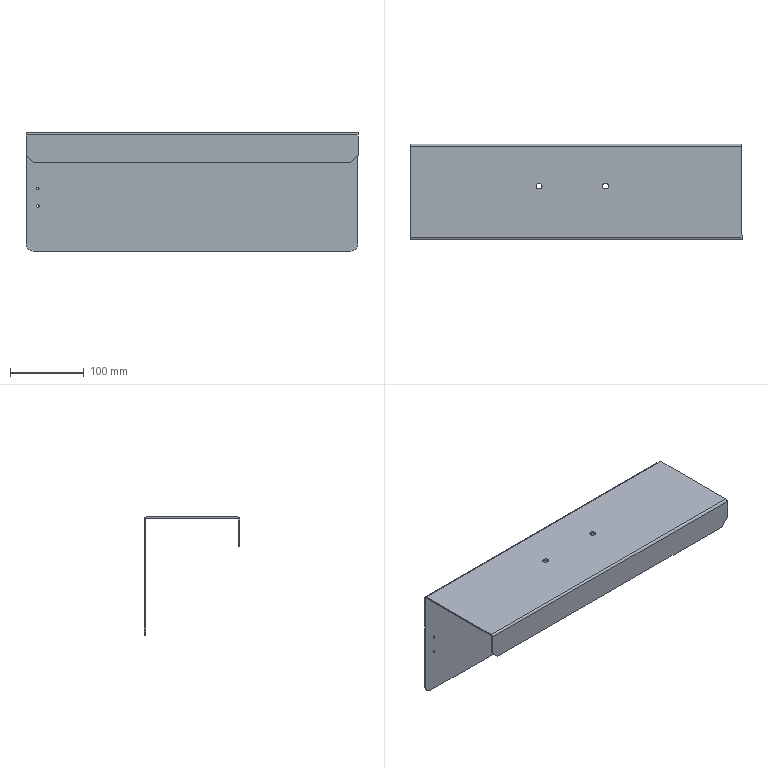Component | SolidWorks | -UpperGuard-1 | 1 solid | 34 faces | box 450 x 130 x 160 mm | volume 291537 mm3 | plane 20 | cylinder 14 | commonest cylinder face diameters 3.3 x4 8 x4 5.473 x2 1.473 x2 20 x2
STEP:
#1=COLOUR_RGB('',0.7922,0.8196,0.9333);
#2=FILL_AREA_STYLE_COLOUR('',#1);
#3=FILL_AREA_STYLE('',(#2));
#4=SURFACE_STYLE_FILL_AREA(#3);
#5=SURFACE_SIDE_STYLE('',(#4));
#6=SURFACE_STYLE_USAGE(.BOTH.,#5);
#7=PRESENTATION_STYLE_ASSIGNMENT((#6));
#8=CARTESIAN_POINT('',(-6.85,51.555,3.951));
#9=VERTEX_POINT('',#8);
#10=CARTESIAN_POINT('',(-6.85,51.555,4.081));
#11=VERTEX_POINT('',#10);
#12=CARTESIAN_POINT('',(-6.85,51.555,4.016));
#13=DIRECTION('',(-0.,1.,0.));
#14=DIRECTION('',(0.,0.,1.));
#15=AXIS2_PLACEMENT_3D('',#12,#13,#14);
#16=CIRCLE('',#15,0.06496);
#17=EDGE_CURVE('',#9,#11,#16,.T.);
#18=ORIENTED_EDGE('',*,*,#17,.F.);
#19=CARTESIAN_POINT('',(-6.85,51.634,3.951));
#20=VERTEX_POINT('',#19);
#21=CARTESIAN_POINT('',(-6.85,51.634,3.951));
#22=DIRECTION('',(-0.,1.,0.));
#23=VECTOR('',#22,39.37);
#24=LINE('',#21,#23);
#25=EDGE_CURVE('',#9,#20,#24,.T.);
#26=ORIENTED_EDGE('',*,*,#25,.T.);
#27=CARTESIAN_POINT('',(-6.85,51.634,4.081));
#28=VERTEX_POINT('',#27);
#29=CARTESIAN_POINT('',(-6.85,51.634,4.016));
#30=DIRECTION('',(-0.,1.,0.));
#31=DIRECTION('',(0.,0.,1.));
#32=AXIS2_PLACEMENT_3D('',#29,#30,#31);
#33=CIRCLE('',#32,0.06496);
#34=EDGE_CURVE('',#20,#28,#33,.T.);
#35=ORIENTED_EDGE('',*,*,#34,.T.);
#36=CARTESIAN_POINT('',(-6.85,51.634,4.081));
#37=DIRECTION('',(-0.,1.,0.));
#38=VECTOR('',#37,39.37);
#39=LINE('',#36,#38);
#40=EDGE_CURVE('',#11,#28,#39,.T.);
#41=ORIENTED_EDGE('',*,*,#40,.F.);
#42=EDGE_LOOP('',(#18,#26,#35,#41));
#43=FACE_OUTER_BOUND('',#42,.T.);
#44=CARTESIAN_POINT('',(-6.85,51.634,4.016));
#45=DIRECTION('',(-0.,1.,0.));
#46=DIRECTION('',(0.,0.,1.));
#47=AXIS2_PLACEMENT_3D('',#44,#45,#46);
#48=CYLINDRICAL_SURFACE('',#47,0.06496);
#49=ADVANCED_FACE('',(#43),#48,.F.);
#50=CARTESIAN_POINT('',(-6.85,51.555,3.006));
#51=VERTEX_POINT('',#50);
#52=CARTESIAN_POINT('',(-6.85,51.555,3.136));
#53=VERTEX_POINT('',#52);
#54=CARTESIAN_POINT('',(-6.85,51.555,3.071));
#55=DIRECTION('',(-0.,1.,0.));
#56=DIRECTION('',(0.,0.,1.));
#57=AXIS2_PLACEMENT_3D('',#54,#55,#56);
#58=CIRCLE('',#57,0.06496);
#59=EDGE_CURVE('',#51,#53,#58,.T.);
#60=ORIENTED_EDGE('',*,*,#59,.F.);
#61=CARTESIAN_POINT('',(-6.85,51.634,3.006));
#62=VERTEX_POINT('',#61);
#63=CARTESIAN_POINT('',(-6.85,51.634,3.006));
#64=DIRECTION('',(-0.,1.,0.));
#65=VECTOR('',#64,39.37);
#66=LINE('',#63,#65);
#67=EDGE_CURVE('',#51,#62,#66,.T.);
#68=ORIENTED_EDGE('',*,*,#67,.T.);
#69=CARTESIAN_POINT('',(-6.85,51.634,3.136));
#70=VERTEX_POINT('',#69);
#71=CARTESIAN_POINT('',(-6.85,51.634,3.071));
#72=DIRECTION('',(-0.,1.,0.));
#73=DIRECTION('',(0.,0.,1.));
#74=AXIS2_PLACEMENT_3D('',#71,#72,#73);
#75=CIRCLE('',#74,0.06496);
#76=EDGE_CURVE('',#62,#70,#75,.T.);
#77=ORIENTED_EDGE('',*,*,#76,.T.);
#78=CARTESIAN_POINT('',(-6.85,51.634,3.136));
#79=DIRECTION('',(-0.,1.,0.));
#80=VECTOR('',#79,39.37);
#81=LINE('',#78,#80);
#82=EDGE_CURVE('',#53,#70,#81,.T.);
#83=ORIENTED_EDGE('',*,*,#82,.F.);
#84=EDGE_LOOP('',(#60,#68,#77,#83));
#85=FACE_OUTER_BOUND('',#84,.T.);
#86=CARTESIAN_POINT('',(-6.85,51.634,3.071));
#87=DIRECTION('',(-0.,1.,0.));
#88=DIRECTION('',(0.,0.,1.));
#89=AXIS2_PLACEMENT_3D('',#86,#87,#88);
#90=CYLINDRICAL_SURFACE('',#89,0.06496);
#91=ADVANCED_FACE('',(#85),#90,.F.);
#92=CARTESIAN_POINT('',(-0.4331,49.39,6.89));
#93=VERTEX_POINT('',#92);
#94=CARTESIAN_POINT('',(-0.748,49.39,6.89));
#95=VERTEX_POINT('',#94);
#96=CARTESIAN_POINT('',(-0.5906,49.39,6.89));
#97=DIRECTION('',(0.,-0.,1.));
#98=DIRECTION('',(-1.,0.,0.));
#99=AXIS2_PLACEMENT_3D('',#96,#97,#98);
#100=CIRCLE('',#99,0.1575);
#101=EDGE_CURVE('',#93,#95,#100,.T.);
#102=ORIENTED_EDGE('',*,*,#101,.F.);
#103=CARTESIAN_POINT('',(-0.4331,49.39,6.969));
#104=VERTEX_POINT('',#103);
#105=CARTESIAN_POINT('',(-0.4331,49.39,6.575));
#106=DIRECTION('',(0.,-0.,1.));
#107=VECTOR('',#106,39.37);
#108=LINE('',#105,#107);
#109=EDGE_CURVE('',#93,#104,#108,.T.);
#110=ORIENTED_EDGE('',*,*,#109,.T.);
#111=CARTESIAN_POINT('',(-0.748,49.39,6.969));
#112=VERTEX_POINT('',#111);
#113=CARTESIAN_POINT('',(-0.5906,49.39,6.969));
#114=DIRECTION('',(0.,-0.,1.));
#115=DIRECTION('',(-1.,0.,0.));
#116=AXIS2_PLACEMENT_3D('',#113,#114,#115);
#117=CIRCLE('',#116,0.1575);
#118=EDGE_CURVE('',#104,#112,#117,.T.);
#119=ORIENTED_EDGE('',*,*,#118,.T.);
#120=CARTESIAN_POINT('',(-0.748,49.39,6.575));
#121=DIRECTION('',(0.,-0.,1.));
#122=VECTOR('',#121,39.37);
#123=LINE('',#120,#122);
#124=EDGE_CURVE('',#95,#112,#123,.T.);
#125=ORIENTED_EDGE('',*,*,#124,.F.);
#126=EDGE_LOOP('',(#102,#110,#119,#125));
#127=FACE_OUTER_BOUND('',#126,.T.);
#128=CARTESIAN_POINT('',(-0.5906,49.39,6.575));
#129=DIRECTION('',(0.,-0.,1.));
#130=DIRECTION('',(-1.,0.,0.));
#131=AXIS2_PLACEMENT_3D('',#128,#129,#130);
#132=CYLINDRICAL_SURFACE('',#131,0.1575);
#133=ADVANCED_FACE('',(#127),#132,.F.);
#134=CARTESIAN_POINT('',(3.11,49.39,6.89));
#135=VERTEX_POINT('',#134);
#136=CARTESIAN_POINT('',(2.795,49.39,6.89));
#137=VERTEX_POINT('',#136);
#138=CARTESIAN_POINT('',(2.953,49.39,6.89));
#139=DIRECTION('',(0.,-0.,1.));
#140=DIRECTION('',(-1.,0.,0.));
#141=AXIS2_PLACEMENT_3D('',#138,#139,#140);
#142=CIRCLE('',#141,0.1575);
#143=EDGE_CURVE('',#135,#137,#142,.T.);
#144=ORIENTED_EDGE('',*,*,#143,.F.);
#145=CARTESIAN_POINT('',(3.11,49.39,6.969));
#146=VERTEX_POINT('',#145);
#147=CARTESIAN_POINT('',(3.11,49.39,6.575));
#148=DIRECTION('',(0.,-0.,1.));
#149=VECTOR('',#148,39.37);
#150=LINE('',#147,#149);
#151=EDGE_CURVE('',#135,#146,#150,.T.);
#152=ORIENTED_EDGE('',*,*,#151,.T.);
#153=CARTESIAN_POINT('',(2.795,49.39,6.969));
#154=VERTEX_POINT('',#153);
#155=CARTESIAN_POINT('',(2.953,49.39,6.969));
#156=DIRECTION('',(0.,-0.,1.));
#157=DIRECTION('',(-1.,0.,0.));
#158=AXIS2_PLACEMENT_3D('',#155,#156,#157);
#159=CIRCLE('',#158,0.1575);
#160=EDGE_CURVE('',#146,#154,#159,.T.);
#161=ORIENTED_EDGE('',*,*,#160,.T.);
#162=CARTESIAN_POINT('',(2.795,49.39,6.575));
#163=DIRECTION('',(0.,-0.,1.));
#164=VECTOR('',#163,39.37);
#165=LINE('',#162,#164);
#166=EDGE_CURVE('',#137,#154,#165,.T.);
#167=ORIENTED_EDGE('',*,*,#166,.F.);
#168=EDGE_LOOP('',(#144,#152,#161,#167));
#169=FACE_OUTER_BOUND('',#168,.T.);
#170=CARTESIAN_POINT('',(2.953,49.39,6.575));
#171=DIRECTION('',(0.,-0.,1.));
#172=DIRECTION('',(-1.,0.,0.));
#173=AXIS2_PLACEMENT_3D('',#170,#171,#172);
#174=CYLINDRICAL_SURFACE('',#173,0.1575);
#175=ADVANCED_FACE('',(#169),#174,.F.);
#176=CARTESIAN_POINT('',(10.236,51.634,6.861));
#177=VERTEX_POINT('',#176);
#178=CARTESIAN_POINT('',(10.236,51.555,6.861));
#179=VERTEX_POINT('',#178);
#180=CARTESIAN_POINT('',(10.236,51.634,6.861));
#181=DIRECTION('',(0.,-1.,-0.));
#182=VECTOR('',#181,39.37);
#183=LINE('',#180,#182);
#184=EDGE_CURVE('',#177,#179,#183,.T.);
#185=ORIENTED_EDGE('',*,*,#184,.F.);
#186=CARTESIAN_POINT('',(10.236,51.526,6.969));
#187=VERTEX_POINT('',#186);
#188=CARTESIAN_POINT('',(10.236,51.526,6.861));
#189=DIRECTION('',(-1.,-0.,-0.));
#190=DIRECTION('',(0.,0.,1.));
#191=AXIS2_PLACEMENT_3D('',#188,#189,#190);
#192=CIRCLE('',#191,0.1077);
#193=EDGE_CURVE('',#187,#177,#192,.T.);
#194=ORIENTED_EDGE('',*,*,#193,.F.);
#195=CARTESIAN_POINT('',(10.236,51.526,6.89));
#196=VERTEX_POINT('',#195);
#197=CARTESIAN_POINT('',(10.236,51.526,6.89));
#198=DIRECTION('',(0.,-0.,1.));
#199=VECTOR('',#198,39.37);
#200=LINE('',#197,#199);
#201=EDGE_CURVE('',#196,#187,#200,.T.);
#202=ORIENTED_EDGE('',*,*,#201,.F.);
#203=CARTESIAN_POINT('',(10.236,51.526,6.861));
#204=DIRECTION('',(-1.,-0.,-0.));
#205=DIRECTION('',(0.,0.,1.));
#206=AXIS2_PLACEMENT_3D('',#203,#204,#205);
#207=CIRCLE('',#206,0.029);
#208=EDGE_CURVE('',#196,#179,#207,.T.);
#209=ORIENTED_EDGE('',*,*,#208,.T.);
#210=EDGE_LOOP('',(#185,#194,#202,#209));
#211=FACE_OUTER_BOUND('',#210,.T.);
#212=CARTESIAN_POINT('',(10.236,51.634,6.861));
#213=DIRECTION('',(1.,0.,-0.));
#214=DIRECTION('',(0.,-0.,1.));
#215=AXIS2_PLACEMENT_3D('',#212,#213,#214);
#216=PLANE('',#215);
#217=ADVANCED_FACE('',(#211),#216,.T.);
#218=CARTESIAN_POINT('',(10.236,51.555,1.063));
#219=VERTEX_POINT('',#218);
#220=CARTESIAN_POINT('',(10.236,51.555,6.969));
#221=DIRECTION('',(-0.,0.,-1.));
#222=VECTOR('',#221,39.37);
#223=LINE('',#220,#222);
#224=EDGE_CURVE('',#179,#219,#223,.T.);
#225=ORIENTED_EDGE('',*,*,#224,.T.);
#226=CARTESIAN_POINT('',(10.236,51.634,1.063));
#227=VERTEX_POINT('',#226);
#228=CARTESIAN_POINT('',(10.236,51.526,1.063));
#229=DIRECTION('',(-0.,1.,0.));
#230=VECTOR('',#229,39.37);
#231=LINE('',#228,#230);
#232=EDGE_CURVE('',#219,#227,#231,.T.);
#233=ORIENTED_EDGE('',*,*,#232,.T.);
#234=CARTESIAN_POINT('',(10.236,51.634,6.969));
#235=DIRECTION('',(-0.,0.,-1.));
#236=VECTOR('',#235,39.37);
#237=LINE('',#234,#236);
#238=EDGE_CURVE('',#177,#227,#237,.T.);
#239=ORIENTED_EDGE('',*,*,#238,.F.);
#240=ORIENTED_EDGE('',*,*,#184,.T.);
#241=EDGE_LOOP('',(#225,#233,#239,#240));
#242=FACE_OUTER_BOUND('',#241,.T.);
#243=CARTESIAN_POINT('',(10.236,51.526,6.89));
#244=DIRECTION('',(1.,0.,-0.));
#245=DIRECTION('',(0.,-0.,1.));
#246=AXIS2_PLACEMENT_3D('',#243,#244,#245);
#247=PLANE('',#246);
#248=ADVANCED_FACE('',(#242),#247,.T.);
#249=CARTESIAN_POINT('',(-7.48,51.526,6.969));
#250=VERTEX_POINT('',#249);
#251=CARTESIAN_POINT('',(-7.48,51.526,6.89));
#252=VERTEX_POINT('',#251);
#253=CARTESIAN_POINT('',(-7.48,51.526,6.969));
#254=DIRECTION('',(-0.,0.,-1.));
#255=VECTOR('',#254,39.37);
#256=LINE('',#253,#255);
#257=EDGE_CURVE('',#250,#252,#256,.T.);
#258=ORIENTED_EDGE('',*,*,#257,.F.);
#259=CARTESIAN_POINT('',(-7.48,51.634,6.861));
#260=VERTEX_POINT('',#259);
#261=CARTESIAN_POINT('',(-7.48,51.526,6.861));
#262=DIRECTION('',(-1.,-0.,-0.));
#263=DIRECTION('',(0.,0.,1.));
#264=AXIS2_PLACEMENT_3D('',#261,#262,#263);
#265=CIRCLE('',#264,0.1077);
#266=EDGE_CURVE('',#250,#260,#265,.T.);
#267=ORIENTED_EDGE('',*,*,#266,.T.);
#268=CARTESIAN_POINT('',(-7.48,51.555,6.861));
#269=VERTEX_POINT('',#268);
#270=CARTESIAN_POINT('',(-7.48,51.555,6.861));
#271=DIRECTION('',(-0.,1.,0.));
#272=VECTOR('',#271,39.37);
#273=LINE('',#270,#272);
#274=EDGE_CURVE('',#269,#260,#273,.T.);
#275=ORIENTED_EDGE('',*,*,#274,.F.);
#276=CARTESIAN_POINT('',(-7.48,51.526,6.861));
#277=DIRECTION('',(-1.,-0.,-0.));
#278=DIRECTION('',(0.,0.,1.));
#279=AXIS2_PLACEMENT_3D('',#276,#277,#278);
#280=CIRCLE('',#279,0.029);
#281=EDGE_CURVE('',#252,#269,#280,.T.);
#282=ORIENTED_EDGE('',*,*,#281,.F.);
#283=EDGE_LOOP('',(#258,#267,#275,#282));
#284=FACE_OUTER_BOUND('',#283,.T.);
#285=CARTESIAN_POINT('',(-7.48,51.526,6.969));
#286=DIRECTION('',(-1.,-0.,0.));
#287=DIRECTION('',(-0.,0.,-1.));
#288=AXIS2_PLACEMENT_3D('',#285,#286,#287);
#289=PLANE('',#288);
#290=ADVANCED_FACE('',(#284),#289,.T.);
#291=CARTESIAN_POINT('',(-7.48,46.623,6.969));
#292=VERTEX_POINT('',#291);
#293=CARTESIAN_POINT('',(-7.48,46.713,6.969));
#294=DIRECTION('',(-0.,1.,0.));
#295=VECTOR('',#294,39.37);
#296=LINE('',#293,#295);
#297=EDGE_CURVE('',#292,#250,#296,.T.);
#298=ORIENTED_EDGE('',*,*,#297,.T.);
#299=ORIENTED_EDGE('',*,*,#257,.T.);
#300=CARTESIAN_POINT('',(-7.48,46.623,6.89));
#301=VERTEX_POINT('',#300);
#302=CARTESIAN_POINT('',(-7.48,46.713,6.89));
#303=DIRECTION('',(-0.,1.,0.));
#304=VECTOR('',#303,39.37);
#305=LINE('',#302,#304);
#306=EDGE_CURVE('',#301,#252,#305,.T.);
#307=ORIENTED_EDGE('',*,*,#306,.F.);
#308=CARTESIAN_POINT('',(-7.48,46.623,6.89));
#309=DIRECTION('',(0.,-0.,1.));
#310=VECTOR('',#309,39.37);
#311=LINE('',#308,#310);
#312=EDGE_CURVE('',#301,#292,#311,.T.);
#313=ORIENTED_EDGE('',*,*,#312,.T.);
#314=EDGE_LOOP('',(#298,#299,#307,#313));
#315=FACE_OUTER_BOUND('',#314,.T.);
#316=CARTESIAN_POINT('',(-7.48,51.555,6.861));
#317=DIRECTION('',(-1.,-0.,0.));
#318=DIRECTION('',(-0.,0.,-1.));
#319=AXIS2_PLACEMENT_3D('',#316,#317,#318);
#320=PLANE('',#319);
#321=ADVANCED_FACE('',(#315),#320,.T.);
#322=CARTESIAN_POINT('',(-6.85,51.555,4.016));
#323=DIRECTION('',(-0.,1.,0.));
#324=DIRECTION('',(0.,0.,1.));
#325=AXIS2_PLACEMENT_3D('',#322,#323,#324);
#326=CIRCLE('',#325,0.06496);
#327=EDGE_CURVE('',#11,#9,#326,.T.);
#328=ORIENTED_EDGE('',*,*,#327,.T.);
#329=ORIENTED_EDGE('',*,*,#17,.T.);
#330=EDGE_LOOP('',(#328,#329));
#331=FACE_BOUND('',#330,.T.);
#332=CARTESIAN_POINT('',(-6.85,51.555,3.071));
#333=DIRECTION('',(-0.,1.,0.));
#334=DIRECTION('',(0.,0.,1.));
#335=AXIS2_PLACEMENT_3D('',#332,#333,#334);
#336=CIRCLE('',#335,0.06496);
#337=EDGE_CURVE('',#53,#51,#336,.T.);
#338=ORIENTED_EDGE('',*,*,#337,.T.);
#339=ORIENTED_EDGE('',*,*,#59,.T.);
#340=EDGE_LOOP('',(#338,#339));
#341=FACE_BOUND('',#340,.T.);
#342=CARTESIAN_POINT('',(-7.48,51.555,1.063));
#343=VERTEX_POINT('',#342);
#344=CARTESIAN_POINT('',(-7.48,51.555,6.969));
#345=DIRECTION('',(-0.,0.,-1.));
#346=VECTOR('',#345,39.37);
#347=LINE('',#344,#346);
#348=EDGE_CURVE('',#269,#343,#347,.T.);
#349=ORIENTED_EDGE('',*,*,#348,.T.);
#350=CARTESIAN_POINT('',(-7.087,51.555,0.6693));
#351=VERTEX_POINT('',#350);
#352=CARTESIAN_POINT('',(-7.087,51.555,1.063));
#353=DIRECTION('',(0.,-1.,-0.));
#354=DIRECTION('',(0.,0.,1.));
#355=AXIS2_PLACEMENT_3D('',#352,#353,#354);
#356=CIRCLE('',#355,0.3937);
#357=EDGE_CURVE('',#343,#351,#356,.T.);
#358=ORIENTED_EDGE('',*,*,#357,.T.);
#359=CARTESIAN_POINT('',(9.843,51.555,0.6693));
#360=VERTEX_POINT('',#359);
#361=CARTESIAN_POINT('',(10.236,51.555,0.6693));
#362=DIRECTION('',(-1.,-0.,-0.));
#363=VECTOR('',#362,39.37);
#364=LINE('',#361,#363);
#365=EDGE_CURVE('',#360,#351,#364,.T.);
#366=ORIENTED_EDGE('',*,*,#365,.F.);
#367=CARTESIAN_POINT('',(9.843,51.555,1.063));
#368=DIRECTION('',(0.,-1.,-0.));
#369=DIRECTION('',(0.,0.,1.));
#370=AXIS2_PLACEMENT_3D('',#367,#368,#369);
#371=CIRCLE('',#370,0.3937);
#372=EDGE_CURVE('',#360,#219,#371,.T.);
#373=ORIENTED_EDGE('',*,*,#372,.T.);
#374=ORIENTED_EDGE('',*,*,#224,.F.);
#375=CARTESIAN_POINT('',(10.236,51.555,6.861));
#376=DIRECTION('',(-1.,-0.,-0.));
#377=VECTOR('',#376,39.37);
#378=LINE('',#375,#377);
#379=EDGE_CURVE('',#179,#269,#378,.T.);
#380=ORIENTED_EDGE('',*,*,#379,.T.);
#381=EDGE_LOOP('',(#349,#358,#366,#373,#374,#380));
#382=FACE_OUTER_BOUND('',#381,.T.);
#383=CARTESIAN_POINT('',(10.236,51.555,6.969));
#384=DIRECTION('',(-0.,1.,0.));
#385=DIRECTION('',(0.,-0.,1.));
#386=AXIS2_PLACEMENT_3D('',#383,#384,#385);
#387=PLANE('',#386);
#388=ADVANCED_FACE('',(#331,#341,#382),#387,.F.);
#389=ORIENTED_EDGE('',*,*,#365,.T.);
#390=CARTESIAN_POINT('',(-7.087,51.634,0.6693));
#391=VERTEX_POINT('',#390);
#392=CARTESIAN_POINT('',(-7.087,51.634,0.6693));
#393=DIRECTION('',(-0.,1.,0.));
#394=VECTOR('',#393,39.37);
#395=LINE('',#392,#394);
#396=EDGE_CURVE('',#351,#391,#395,.T.);
#397=ORIENTED_EDGE('',*,*,#396,.T.);
#398=CARTESIAN_POINT('',(9.843,51.634,0.6693));
#399=VERTEX_POINT('',#398);
#400=CARTESIAN_POINT('',(10.236,51.634,0.6693));
#401=DIRECTION('',(-1.,-0.,-0.));
#402=VECTOR('',#401,39.37);
#403=LINE('',#400,#402);
#404=EDGE_CURVE('',#399,#391,#403,.T.);
#405=ORIENTED_EDGE('',*,*,#404,.F.);
#406=CARTESIAN_POINT('',(9.843,51.634,0.6693));
#407=DIRECTION('',(0.,-1.,-0.));
#408=VECTOR('',#407,39.37);
#409=LINE('',#406,#408);
#410=EDGE_CURVE('',#399,#360,#409,.T.);
#411=ORIENTED_EDGE('',*,*,#410,.T.);
#412=EDGE_LOOP('',(#389,#397,#405,#411));
#413=FACE_OUTER_BOUND('',#412,.T.);
#414=CARTESIAN_POINT('',(10.236,51.634,0.6693));
#415=DIRECTION('',(0.,0.,-1.));
#416=DIRECTION('',(1.,0.,0.));
#417=AXIS2_PLACEMENT_3D('',#414,#415,#416);
#418=PLANE('',#417);
#419=ADVANCED_FACE('',(#413),#418,.T.);
#420=CARTESIAN_POINT('',(-6.85,51.634,4.016));
#421=DIRECTION('',(-0.,1.,0.));
#422=DIRECTION('',(0.,0.,1.));
#423=AXIS2_PLACEMENT_3D('',#420,#421,#422);
#424=CIRCLE('',#423,0.06496);
#425=EDGE_CURVE('',#28,#20,#424,.T.);
#426=ORIENTED_EDGE('',*,*,#425,.F.);
#427=ORIENTED_EDGE('',*,*,#34,.F.);
#428=EDGE_LOOP('',(#426,#427));
#429=FACE_BOUND('',#428,.T.);
#430=CARTESIAN_POINT('',(-6.85,51.634,3.071));
#431=DIRECTION('',(-0.,1.,0.));
#432=DIRECTION('',(0.,0.,1.));
#433=AXIS2_PLACEMENT_3D('',#430,#431,#432);
#434=CIRCLE('',#433,0.06496);
#435=EDGE_CURVE('',#70,#62,#434,.T.);
#436=ORIENTED_EDGE('',*,*,#435,.F.);
#437=ORIENTED_EDGE('',*,*,#76,.F.);
#438=EDGE_LOOP('',(#436,#437));
#439=FACE_BOUND('',#438,.T.);
#440=ORIENTED_EDGE('',*,*,#404,.T.);
#441=CARTESIAN_POINT('',(-7.48,51.634,1.063));
#442=VERTEX_POINT('',#441);
#443=CARTESIAN_POINT('',(-7.087,51.634,1.063));
#444=DIRECTION('',(-0.,1.,0.));
#445=DIRECTION('',(0.,0.,1.));
#446=AXIS2_PLACEMENT_3D('',#443,#444,#445);
#447=CIRCLE('',#446,0.3937);
#448=EDGE_CURVE('',#391,#442,#447,.T.);
#449=ORIENTED_EDGE('',*,*,#448,.T.);
#450=CARTESIAN_POINT('',(-7.48,51.634,6.969));
#451=DIRECTION('',(-0.,0.,-1.));
#452=VECTOR('',#451,39.37);
#453=LINE('',#450,#452);
#454=EDGE_CURVE('',#260,#442,#453,.T.);
#455=ORIENTED_EDGE('',*,*,#454,.F.);
#456=CARTESIAN_POINT('',(10.236,51.634,6.861));
#457=DIRECTION('',(-1.,-0.,-0.));
#458=VECTOR('',#457,39.37);
#459=LINE('',#456,#458);
#460=EDGE_CURVE('',#177,#260,#459,.T.);
#461=ORIENTED_EDGE('',*,*,#460,.F.);
#462=ORIENTED_EDGE('',*,*,#238,.T.);
#463=CARTESIAN_POINT('',(9.843,51.634,1.063));
#464=DIRECTION('',(-0.,1.,0.));
#465=DIRECTION('',(0.,0.,1.));
#466=AXIS2_PLACEMENT_3D('',#463,#464,#465);
#467=CIRCLE('',#466,0.3937);
#468=EDGE_CURVE('',#227,#399,#467,.T.);
#469=ORIENTED_EDGE('',*,*,#468,.T.);
#470=EDGE_LOOP('',(#440,#449,#455,#461,#462,#469));
#471=FACE_OUTER_BOUND('',#470,.T.);
#472=CARTESIAN_POINT('',(10.236,51.634,6.969));
#473=DIRECTION('',(-0.,1.,0.));
#474=DIRECTION('',(0.,-0.,1.));
#475=AXIS2_PLACEMENT_3D('',#472,#473,#474);
#476=PLANE('',#475);
#477=ADVANCED_FACE('',(#429,#439,#471),#476,.T.);
#478=ORIENTED_EDGE('',*,*,#266,.F.);
#479=CARTESIAN_POINT('',(10.236,51.526,6.969));
#480=DIRECTION('',(-1.,-0.,-0.));
#481=VECTOR('',#480,39.37);
#482=LINE('',#479,#481);
#483=EDGE_CURVE('',#187,#250,#482,.T.);
#484=ORIENTED_EDGE('',*,*,#483,.F.);
#485=ORIENTED_EDGE('',*,*,#193,.T.);
#486=ORIENTED_EDGE('',*,*,#460,.T.);
#487=EDGE_LOOP('',(#478,#484,#485,#486));
#488=FACE_OUTER_BOUND('',#487,.T.);
#489=CARTESIAN_POINT('',(10.236,51.526,6.861));
#490=DIRECTION('',(-1.,-0.,-0.));
#491=DIRECTION('',(0.,0.,-1.));
#492=AXIS2_PLACEMENT_3D('',#489,#490,#491);
#493=CYLINDRICAL_SURFACE('',#492,0.1077);
#494=ADVANCED_FACE('',(#488),#493,.T.);
#495=CARTESIAN_POINT('',(-0.5906,49.39,6.969));
#496=DIRECTION('',(0.,-0.,1.));
#497=DIRECTION('',(-1.,0.,0.));
#498=AXIS2_PLACEMENT_3D('',#495,#496,#497);
#499=CIRCLE('',#498,0.1575);
#500=EDGE_CURVE('',#112,#104,#499,.T.);
#501=ORIENTED_EDGE('',*,*,#500,.F.);
#502=ORIENTED_EDGE('',*,*,#118,.F.);
#503=EDGE_LOOP('',(#501,#502));
#504=FACE_BOUND('',#503,.T.);
#505=CARTESIAN_POINT('',(2.953,49.39,6.969));
#506=DIRECTION('',(0.,-0.,1.));
#507=DIRECTION('',(-1.,0.,0.));
#508=AXIS2_PLACEMENT_3D('',#505,#506,#507);
#509=CIRCLE('',#508,0.1575);
#510=EDGE_CURVE('',#154,#146,#509,.T.);
#511=ORIENTED_EDGE('',*,*,#510,.F.);
#512=ORIENTED_EDGE('',*,*,#160,.F.);
#513=EDGE_LOOP('',(#511,#512));
#514=FACE_BOUND('',#513,.T.);
#515=ORIENTED_EDGE('',*,*,#297,.F.);
#516=CARTESIAN_POINT('',(10.236,46.623,6.969));
#517=VERTEX_POINT('',#516);
#518=CARTESIAN_POINT('',(-7.48,46.623,6.969));
#519=DIRECTION('',(1.,0.,0.));
#520=VECTOR('',#519,39.37);
#521=LINE('',#518,#520);
#522=EDGE_CURVE('',#292,#517,#521,.T.);
#523=ORIENTED_EDGE('',*,*,#522,.T.);
#524=CARTESIAN_POINT('',(10.236,46.713,6.969));
#525=DIRECTION('',(-0.,1.,0.));
#526=VECTOR('',#525,39.37);
#527=LINE('',#524,#526);
#528=EDGE_CURVE('',#517,#187,#527,.T.);
#529=ORIENTED_EDGE('',*,*,#528,.T.);
#530=ORIENTED_EDGE('',*,*,#483,.T.);
#531=EDGE_LOOP('',(#515,#523,#529,#530));
#532=FACE_OUTER_BOUND('',#531,.T.);
#533=CARTESIAN_POINT('',(10.236,46.713,6.969));
#534=DIRECTION('',(-0.,-0.,1.));
#535=DIRECTION('',(-1.,-0.,-0.));
#536=AXIS2_PLACEMENT_3D('',#533,#534,#535);
#537=PLANE('',#536);
#538=ADVANCED_FACE('',(#504,#514,#532),#537,.T.);
#539=CARTESIAN_POINT('',(-0.5906,49.39,6.89));
#540=DIRECTION('',(0.,-0.,1.));
#541=DIRECTION('',(-1.,0.,0.));
#542=AXIS2_PLACEMENT_3D('',#539,#540,#541);
#543=CIRCLE('',#542,0.1575);
#544=EDGE_CURVE('',#95,#93,#543,.T.);
#545=ORIENTED_EDGE('',*,*,#544,.T.);
#546=ORIENTED_EDGE('',*,*,#101,.T.);
#547=EDGE_LOOP('',(#545,#546));
#548=FACE_BOUND('',#547,.T.);
#549=CARTESIAN_POINT('',(2.953,49.39,6.89));
#550=DIRECTION('',(0.,-0.,1.));
#551=DIRECTION('',(-1.,0.,0.));
#552=AXIS2_PLACEMENT_3D('',#549,#550,#551);
#553=CIRCLE('',#552,0.1575);
#554=EDGE_CURVE('',#137,#135,#553,.T.);
#555=ORIENTED_EDGE('',*,*,#554,.T.);
#556=ORIENTED_EDGE('',*,*,#143,.T.);
#557=EDGE_LOOP('',(#555,#556));
#558=FACE_BOUND('',#557,.T.);
#559=ORIENTED_EDGE('',*,*,#306,.T.);
#560=CARTESIAN_POINT('',(10.236,51.526,6.89));
#561=DIRECTION('',(-1.,-0.,-0.));
#562=VECTOR('',#561,39.37);
#563=LINE('',#560,#562);
#564=EDGE_CURVE('',#196,#252,#563,.T.);
#565=ORIENTED_EDGE('',*,*,#564,.F.);
#566=CARTESIAN_POINT('',(10.236,46.623,6.89));
#567=VERTEX_POINT('',#566);
#568=CARTESIAN_POINT('',(10.236,46.713,6.89));
#569=DIRECTION('',(-0.,1.,0.));
#570=VECTOR('',#569,39.37);
#571=LINE('',#568,#570);
#572=EDGE_CURVE('',#567,#196,#571,.T.);
#573=ORIENTED_EDGE('',*,*,#572,.F.);
#574=CARTESIAN_POINT('',(-7.48,46.623,6.89));
#575=DIRECTION('',(1.,0.,0.));
#576=VECTOR('',#575,39.37);
#577=LINE('',#574,#576);
#578=EDGE_CURVE('',#301,#567,#577,.T.);
#579=ORIENTED_EDGE('',*,*,#578,.F.);
#580=EDGE_LOOP('',(#559,#565,#573,#579));
#581=FACE_OUTER_BOUND('',#580,.T.);
#582=CARTESIAN_POINT('',(10.236,46.713,6.89));
#583=DIRECTION('',(-0.,-0.,1.));
#584=DIRECTION('',(-1.,-0.,-0.));
#585=AXIS2_PLACEMENT_3D('',#582,#583,#584);
#586=PLANE('',#585);
#587=ADVANCED_FACE('',(#548,#558,#581),#586,.F.);
#588=ORIENTED_EDGE('',*,*,#281,.T.);
#589=ORIENTED_EDGE('',*,*,#379,.F.);
#590=ORIENTED_EDGE('',*,*,#208,.F.);
#591=ORIENTED_EDGE('',*,*,#564,.T.);
#592=EDGE_LOOP('',(#588,#589,#590,#591));
#593=FACE_OUTER_BOUND('',#592,.T.);
#594=CARTESIAN_POINT('',(10.236,51.526,6.861));
#595=DIRECTION('',(-1.,-0.,-0.));
#596=DIRECTION('',(0.,0.,-1.));
#597=AXIS2_PLACEMENT_3D('',#594,#595,#596);
#598=CYLINDRICAL_SURFACE('',#597,0.029);
#599=ADVANCED_FACE('',(#593),#598,.F.);
#600=ORIENTED_EDGE('',*,*,#572,.T.);
#601=ORIENTED_EDGE('',*,*,#201,.T.);
#602=ORIENTED_EDGE('',*,*,#528,.F.);
#603=CARTESIAN_POINT('',(10.236,46.623,6.89));
#604=DIRECTION('',(0.,-0.,1.));
#605=VECTOR('',#604,39.37);
#606=LINE('',#603,#605);
#607=EDGE_CURVE('',#567,#517,#606,.T.);
#608=ORIENTED_EDGE('',*,*,#607,.F.);
#609=EDGE_LOOP('',(#600,#601,#602,#608));
#610=FACE_OUTER_BOUND('',#609,.T.);
#611=CARTESIAN_POINT('',(10.236,51.526,6.861));
#612=DIRECTION('',(1.,0.,-0.));
#613=DIRECTION('',(0.,-0.,1.));
#614=AXIS2_PLACEMENT_3D('',#611,#612,#613);
#615=PLANE('',#614);
#616=ADVANCED_FACE('',(#610),#615,.T.);
#617=ORIENTED_EDGE('',*,*,#454,.T.);
#618=CARTESIAN_POINT('',(-7.48,51.555,1.063));
#619=DIRECTION('',(0.,-1.,-0.));
#620=VECTOR('',#619,39.37);
#621=LINE('',#618,#620);
#622=EDGE_CURVE('',#442,#343,#621,.T.);
#623=ORIENTED_EDGE('',*,*,#622,.T.);
#624=ORIENTED_EDGE('',*,*,#348,.F.);
#625=ORIENTED_EDGE('',*,*,#274,.T.);
#626=EDGE_LOOP('',(#617,#623,#624,#625));
#627=FACE_OUTER_BOUND('',#626,.T.);
#628=CARTESIAN_POINT('',(-7.48,51.526,6.861));
#629=DIRECTION('',(1.,0.,-0.));
#630=DIRECTION('',(0.,-0.,1.));
#631=AXIS2_PLACEMENT_3D('',#628,#629,#630);
#632=PLANE('',#631);
#633=ADVANCED_FACE('',(#627),#632,.F.);
#634=ORIENTED_EDGE('',*,*,#151,.F.);
#635=ORIENTED_EDGE('',*,*,#554,.F.);
#636=ORIENTED_EDGE('',*,*,#166,.T.);
#637=ORIENTED_EDGE('',*,*,#510,.T.);
#638=EDGE_LOOP('',(#634,#635,#636,#637));
#639=FACE_OUTER_BOUND('',#638,.T.);
#640=CARTESIAN_POINT('',(2.953,49.39,6.575));
#641=DIRECTION('',(0.,-0.,1.));
#642=DIRECTION('',(-1.,0.,0.));
#643=AXIS2_PLACEMENT_3D('',#640,#641,#642);
#644=CYLINDRICAL_SURFACE('',#643,0.1575);
#645=ADVANCED_FACE('',(#639),#644,.F.);
#646=ORIENTED_EDGE('',*,*,#109,.F.);
#647=ORIENTED_EDGE('',*,*,#544,.F.);
#648=ORIENTED_EDGE('',*,*,#124,.T.);
#649=ORIENTED_EDGE('',*,*,#500,.T.);
#650=EDGE_LOOP('',(#646,#647,#648,#649));
#651=FACE_OUTER_BOUND('',#650,.T.);
#652=CARTESIAN_POINT('',(-0.5906,49.39,6.575));
#653=DIRECTION('',(0.,-0.,1.));
#654=DIRECTION('',(-1.,0.,0.));
#655=AXIS2_PLACEMENT_3D('',#652,#653,#654);
#656=CYLINDRICAL_SURFACE('',#655,0.1575);
#657=ADVANCED_FACE('',(#651),#656,.F.);
#658=ORIENTED_EDGE('',*,*,#448,.F.);
#659=ORIENTED_EDGE('',*,*,#396,.F.);
#660=ORIENTED_EDGE('',*,*,#357,.F.);
#661=ORIENTED_EDGE('',*,*,#622,.F.);
#662=EDGE_LOOP('',(#658,#659,#660,#661));
#663=FACE_OUTER_BOUND('',#662,.T.);
#664=CARTESIAN_POINT('',(-7.087,51.526,1.063));
#665=DIRECTION('',(-0.,1.,0.));
#666=DIRECTION('',(0.,0.,1.));
#667=AXIS2_PLACEMENT_3D('',#664,#665,#666);
#668=CYLINDRICAL_SURFACE('',#667,0.3937);
#669=ADVANCED_FACE('',(#663),#668,.T.);
#670=ORIENTED_EDGE('',*,*,#468,.F.);
#671=ORIENTED_EDGE('',*,*,#232,.F.);
#672=ORIENTED_EDGE('',*,*,#372,.F.);
#673=ORIENTED_EDGE('',*,*,#410,.F.);
#674=EDGE_LOOP('',(#670,#671,#672,#673));
#675=FACE_OUTER_BOUND('',#674,.T.);
#676=CARTESIAN_POINT('',(9.843,51.634,1.063));
#677=DIRECTION('',(0.,-1.,-0.));
#678=DIRECTION('',(0.,0.,-1.));
#679=AXIS2_PLACEMENT_3D('',#676,#677,#678);
#680=CYLINDRICAL_SURFACE('',#679,0.3937);
#681=ADVANCED_FACE('',(#675),#680,.T.);
#682=ORIENTED_EDGE('',*,*,#67,.F.);
#683=ORIENTED_EDGE('',*,*,#337,.F.);
#684=ORIENTED_EDGE('',*,*,#82,.T.);
#685=ORIENTED_EDGE('',*,*,#435,.T.);
#686=EDGE_LOOP('',(#682,#683,#684,#685));
#687=FACE_OUTER_BOUND('',#686,.T.);
#688=CARTESIAN_POINT('',(-6.85,51.634,3.071));
#689=DIRECTION('',(-0.,1.,0.));
#690=DIRECTION('',(0.,0.,1.));
#691=AXIS2_PLACEMENT_3D('',#688,#689,#690);
#692=CYLINDRICAL_SURFACE('',#691,0.06496);
#693=ADVANCED_FACE('',(#687),#692,.F.);
#694=ORIENTED_EDGE('',*,*,#25,.F.);
#695=ORIENTED_EDGE('',*,*,#327,.F.);
#696=ORIENTED_EDGE('',*,*,#40,.T.);
#697=ORIENTED_EDGE('',*,*,#425,.T.);
#698=EDGE_LOOP('',(#694,#695,#696,#697));
#699=FACE_OUTER_BOUND('',#698,.T.);
#700=CARTESIAN_POINT('',(-6.85,51.634,4.016));
#701=DIRECTION('',(-0.,1.,0.));
#702=DIRECTION('',(0.,0.,1.));
#703=AXIS2_PLACEMENT_3D('',#700,#701,#702);
#704=CYLINDRICAL_SURFACE('',#703,0.06496);
#705=ADVANCED_FACE('',(#699),#704,.F.);
#706=CARTESIAN_POINT('',(10.236,46.594,6.861));
#707=VERTEX_POINT('',#706);
#708=CARTESIAN_POINT('',(10.236,46.516,6.861));
#709=VERTEX_POINT('',#708);
#710=CARTESIAN_POINT('',(10.236,46.516,6.861));
#711=DIRECTION('',(0.,-1.,0.));
#712=VECTOR('',#711,39.37);
#713=LINE('',#710,#712);
#714=EDGE_CURVE('',#707,#709,#713,.T.);
#715=ORIENTED_EDGE('',*,*,#714,.F.);
#716=CARTESIAN_POINT('',(10.236,46.623,6.861));
#717=DIRECTION('',(1.,0.,0.));
#718=DIRECTION('',(0.,0.,-1.));
#719=AXIS2_PLACEMENT_3D('',#716,#717,#718);
#720=CIRCLE('',#719,0.029);
#721=EDGE_CURVE('',#567,#707,#720,.T.);
#722=ORIENTED_EDGE('',*,*,#721,.F.);
#723=ORIENTED_EDGE('',*,*,#607,.T.);
#724=CARTESIAN_POINT('',(10.236,46.623,6.861));
#725=DIRECTION('',(1.,0.,0.));
#726=DIRECTION('',(0.,0.,-1.));
#727=AXIS2_PLACEMENT_3D('',#724,#725,#726);
#728=CIRCLE('',#727,0.1077);
#729=EDGE_CURVE('',#517,#709,#728,.T.);
#730=ORIENTED_EDGE('',*,*,#729,.T.);
#731=EDGE_LOOP('',(#715,#722,#723,#730));
#732=FACE_OUTER_BOUND('',#731,.T.);
#733=CARTESIAN_POINT('',(10.236,46.623,6.861));
#734=DIRECTION('',(1.,0.,-0.));
#735=DIRECTION('',(0.,-0.,1.));
#736=AXIS2_PLACEMENT_3D('',#733,#734,#735);
#737=PLANE('',#736);
#738=ADVANCED_FACE('',(#732),#737,.T.);
#739=CARTESIAN_POINT('',(-7.48,46.594,6.861));
#740=VERTEX_POINT('',#739);
#741=CARTESIAN_POINT('',(-7.48,46.623,6.861));
#742=DIRECTION('',(-1.,-0.,-0.));
#743=DIRECTION('',(0.,0.,-1.));
#744=AXIS2_PLACEMENT_3D('',#741,#742,#743);
#745=CIRCLE('',#744,0.029);
#746=EDGE_CURVE('',#740,#301,#745,.T.);
#747=ORIENTED_EDGE('',*,*,#746,.F.);
#748=CARTESIAN_POINT('',(-7.48,46.516,6.861));
#749=VERTEX_POINT('',#748);
#750=CARTESIAN_POINT('',(-7.48,46.594,6.861));
#751=DIRECTION('',(0.,-1.,0.));
#752=VECTOR('',#751,39.37);
#753=LINE('',#750,#752);
#754=EDGE_CURVE('',#740,#749,#753,.T.);
#755=ORIENTED_EDGE('',*,*,#754,.T.);
#756=CARTESIAN_POINT('',(-7.48,46.623,6.861));
#757=DIRECTION('',(-1.,-0.,-0.));
#758=DIRECTION('',(0.,0.,-1.));
#759=AXIS2_PLACEMENT_3D('',#756,#757,#758);
#760=CIRCLE('',#759,0.1077);
#761=EDGE_CURVE('',#749,#292,#760,.T.);
#762=ORIENTED_EDGE('',*,*,#761,.T.);
#763=ORIENTED_EDGE('',*,*,#312,.F.);
#764=EDGE_LOOP('',(#747,#755,#762,#763));
#765=FACE_OUTER_BOUND('',#764,.T.);
#766=CARTESIAN_POINT('',(-7.48,46.623,6.861));
#767=DIRECTION('',(1.,0.,-0.));
#768=DIRECTION('',(0.,-0.,1.));
#769=AXIS2_PLACEMENT_3D('',#766,#767,#768);
#770=PLANE('',#769);
#771=ADVANCED_FACE('',(#765),#770,.F.);
#772=ORIENTED_EDGE('',*,*,#522,.F.);
#773=ORIENTED_EDGE('',*,*,#761,.F.);
#774=CARTESIAN_POINT('',(1.378,46.516,6.861));
#775=DIRECTION('',(-1.,-0.,-0.));
#776=VECTOR('',#775,39.37);
#777=LINE('',#774,#776);
#778=EDGE_CURVE('',#709,#749,#777,.T.);
#779=ORIENTED_EDGE('',*,*,#778,.F.);
#780=ORIENTED_EDGE('',*,*,#729,.F.);
#781=EDGE_LOOP('',(#772,#773,#779,#780));
#782=FACE_OUTER_BOUND('',#781,.T.);
#783=CARTESIAN_POINT('',(-7.48,46.623,6.861));
#784=DIRECTION('',(-1.,-0.,-0.));
#785=DIRECTION('',(0.,-1.,0.));
#786=AXIS2_PLACEMENT_3D('',#783,#784,#785);
#787=CYLINDRICAL_SURFACE('',#786,0.1077);
#788=ADVANCED_FACE('',(#782),#787,.T.);
#789=ORIENTED_EDGE('',*,*,#578,.T.);
#790=ORIENTED_EDGE('',*,*,#721,.T.);
#791=CARTESIAN_POINT('',(10.236,46.594,6.861));
#792=DIRECTION('',(-1.,-0.,-0.));
#793=VECTOR('',#792,39.37);
#794=LINE('',#791,#793);
#795=EDGE_CURVE('',#707,#740,#794,.T.);
#796=ORIENTED_EDGE('',*,*,#795,.T.);
#797=ORIENTED_EDGE('',*,*,#746,.T.);
#798=EDGE_LOOP('',(#789,#790,#796,#797));
#799=FACE_OUTER_BOUND('',#798,.T.);
#800=CARTESIAN_POINT('',(-7.48,46.623,6.861));
#801=DIRECTION('',(-1.,-0.,-0.));
#802=DIRECTION('',(0.,-1.,0.));
#803=AXIS2_PLACEMENT_3D('',#800,#801,#802);
#804=CYLINDRICAL_SURFACE('',#803,0.029);
#805=ADVANCED_FACE('',(#799),#804,.F.);
#806=CARTESIAN_POINT('',(-7.48,46.594,5.787));
#807=VERTEX_POINT('',#806);
#808=CARTESIAN_POINT('',(-7.48,46.594,6.969));
#809=DIRECTION('',(0.,0.,1.));
#810=VECTOR('',#809,39.37);
#811=LINE('',#808,#810);
#812=EDGE_CURVE('',#807,#740,#811,.T.);
#813=ORIENTED_EDGE('',*,*,#812,.F.);
#814=CARTESIAN_POINT('',(-7.48,46.516,5.787));
#815=VERTEX_POINT('',#814);
#816=CARTESIAN_POINT('',(-7.48,46.516,5.787));
#817=DIRECTION('',(0.,-1.,0.));
#818=VECTOR('',#817,39.37);
#819=LINE('',#816,#818);
#820=EDGE_CURVE('',#807,#815,#819,.T.);
#821=ORIENTED_EDGE('',*,*,#820,.T.);
#822=CARTESIAN_POINT('',(-7.48,46.516,6.89));
#823=DIRECTION('',(0.,0.,1.));
#824=VECTOR('',#823,39.37);
#825=LINE('',#822,#824);
#826=EDGE_CURVE('',#815,#749,#825,.T.);
#827=ORIENTED_EDGE('',*,*,#826,.T.);
#828=ORIENTED_EDGE('',*,*,#754,.F.);
#829=EDGE_LOOP('',(#813,#821,#827,#828));
#830=FACE_OUTER_BOUND('',#829,.T.);
#831=CARTESIAN_POINT('',(-7.48,46.516,6.89));
#832=DIRECTION('',(-1.,-0.,0.));
#833=DIRECTION('',(-0.,0.,-1.));
#834=AXIS2_PLACEMENT_3D('',#831,#832,#833);
#835=PLANE('',#834);
#836=ADVANCED_FACE('',(#830),#835,.T.);
#837=CARTESIAN_POINT('',(10.236,46.516,5.787));
#838=VERTEX_POINT('',#837);
#839=CARTESIAN_POINT('',(10.236,46.516,5.394));
#840=DIRECTION('',(-0.,-0.,-1.));
#841=VECTOR('',#840,39.37);
#842=LINE('',#839,#841);
#843=EDGE_CURVE('',#709,#838,#842,.T.);
#844=ORIENTED_EDGE('',*,*,#843,.T.);
#845=CARTESIAN_POINT('',(10.236,46.594,5.787));
#846=VERTEX_POINT('',#845);
#847=CARTESIAN_POINT('',(10.236,46.516,5.787));
#848=DIRECTION('',(-0.,1.,-0.));
#849=VECTOR('',#848,39.37);
#850=LINE('',#847,#849);
#851=EDGE_CURVE('',#838,#846,#850,.T.);
#852=ORIENTED_EDGE('',*,*,#851,.T.);
#853=CARTESIAN_POINT('',(10.236,46.594,6.969));
#854=DIRECTION('',(-0.,-0.,-1.));
#855=VECTOR('',#854,39.37);
#856=LINE('',#853,#855);
#857=EDGE_CURVE('',#707,#846,#856,.T.);
#858=ORIENTED_EDGE('',*,*,#857,.F.);
#859=ORIENTED_EDGE('',*,*,#714,.T.);
#860=EDGE_LOOP('',(#844,#852,#858,#859));
#861=FACE_OUTER_BOUND('',#860,.T.);
#862=CARTESIAN_POINT('',(10.236,46.516,5.394));
#863=DIRECTION('',(1.,0.,-0.));
#864=DIRECTION('',(0.,-0.,1.));
#865=AXIS2_PLACEMENT_3D('',#862,#863,#864);
#866=PLANE('',#865);
#867=ADVANCED_FACE('',(#861),#866,.T.);
#868=CARTESIAN_POINT('',(9.843,46.516,5.394));
#869=VERTEX_POINT('',#868);
#870=CARTESIAN_POINT('',(-7.087,46.516,5.394));
#871=VERTEX_POINT('',#870);
#872=CARTESIAN_POINT('',(-7.48,46.516,5.394));
#873=DIRECTION('',(-1.,-0.,-0.));
#874=VECTOR('',#873,39.37);
#875=LINE('',#872,#874);
#876=EDGE_CURVE('',#869,#871,#875,.T.);
#877=ORIENTED_EDGE('',*,*,#876,.F.);
#878=CARTESIAN_POINT('',(6.398,46.516,1.949));
#879=DIRECTION('',(0.7071,0.,0.7071));
#880=VECTOR('',#879,39.37);
#881=LINE('',#878,#880);
#882=EDGE_CURVE('',#869,#838,#881,.T.);
#883=ORIENTED_EDGE('',*,*,#882,.T.);
#884=ORIENTED_EDGE('',*,*,#843,.F.);
#885=ORIENTED_EDGE('',*,*,#778,.T.);
#886=ORIENTED_EDGE('',*,*,#826,.F.);
#887=CARTESIAN_POINT('',(-3.642,46.516,1.949));
#888=DIRECTION('',(0.7071,0.,-0.7071));
#889=VECTOR('',#888,39.37);
#890=LINE('',#887,#889);
#891=EDGE_CURVE('',#815,#871,#890,.T.);
#892=ORIENTED_EDGE('',*,*,#891,.T.);
#893=EDGE_LOOP('',(#877,#883,#884,#885,#886,#892));
#894=FACE_OUTER_BOUND('',#893,.T.);
#895=CARTESIAN_POINT('',(1.378,46.516,6.969));
#896=DIRECTION('',(0.,-1.,0.));
#897=DIRECTION('',(-0.,-0.,-1.));
#898=AXIS2_PLACEMENT_3D('',#895,#896,#897);
#899=PLANE('',#898);
#900=ADVANCED_FACE('',(#894),#899,.T.);
#901=ORIENTED_EDGE('',*,*,#857,.T.);
#902=CARTESIAN_POINT('',(9.843,46.594,5.394));
#903=VERTEX_POINT('',#902);
#904=CARTESIAN_POINT('',(10.236,46.594,5.787));
#905=DIRECTION('',(-0.7071,-0.,-0.7071));
#906=VECTOR('',#905,39.37);
#907=LINE('',#904,#906);
#908=EDGE_CURVE('',#846,#903,#907,.T.);
#909=ORIENTED_EDGE('',*,*,#908,.T.);
#910=CARTESIAN_POINT('',(-7.087,46.594,5.394));
#911=VERTEX_POINT('',#910);
#912=CARTESIAN_POINT('',(1.378,46.594,5.394));
#913=DIRECTION('',(-1.,-0.,-0.));
#914=VECTOR('',#913,39.37);
#915=LINE('',#912,#914);
#916=EDGE_CURVE('',#903,#911,#915,.T.);
#917=ORIENTED_EDGE('',*,*,#916,.T.);
#918=CARTESIAN_POINT('',(-7.087,46.594,5.394));
#919=DIRECTION('',(-0.7071,-0.,0.7071));
#920=VECTOR('',#919,39.37);
#921=LINE('',#918,#920);
#922=EDGE_CURVE('',#911,#807,#921,.T.);
#923=ORIENTED_EDGE('',*,*,#922,.T.);
#924=ORIENTED_EDGE('',*,*,#812,.T.);
#925=ORIENTED_EDGE('',*,*,#795,.F.);
#926=EDGE_LOOP('',(#901,#909,#917,#923,#924,#925));
#927=FACE_OUTER_BOUND('',#926,.T.);
#928=CARTESIAN_POINT('',(1.378,46.594,6.969));
#929=DIRECTION('',(0.,-1.,0.));
#930=DIRECTION('',(-0.,-0.,-1.));
#931=AXIS2_PLACEMENT_3D('',#928,#929,#930);
#932=PLANE('',#931);
#933=ADVANCED_FACE('',(#927),#932,.F.);
#934=ORIENTED_EDGE('',*,*,#916,.F.);
#935=CARTESIAN_POINT('',(9.843,46.516,5.394));
#936=DIRECTION('',(0.,-1.,0.));
#937=VECTOR('',#936,39.37);
#938=LINE('',#935,#937);
#939=EDGE_CURVE('',#903,#869,#938,.T.);
#940=ORIENTED_EDGE('',*,*,#939,.T.);
#941=ORIENTED_EDGE('',*,*,#876,.T.);
#942=CARTESIAN_POINT('',(-7.087,46.516,5.394));
#943=DIRECTION('',(-0.,1.,-0.));
#944=VECTOR('',#943,39.37);
#945=LINE('',#942,#944);
#946=EDGE_CURVE('',#871,#911,#945,.T.);
#947=ORIENTED_EDGE('',*,*,#946,.T.);
#948=EDGE_LOOP('',(#934,#940,#941,#947));
#949=FACE_OUTER_BOUND('',#948,.T.);
#950=CARTESIAN_POINT('',(-7.48,46.516,5.394));
#951=DIRECTION('',(-0.,-0.,-1.));
#952=DIRECTION('',(-0.,1.,-0.));
#953=AXIS2_PLACEMENT_3D('',#950,#951,#952);
#954=PLANE('',#953);
#955=ADVANCED_FACE('',(#949),#954,.T.);
#956=ORIENTED_EDGE('',*,*,#882,.F.);
#957=ORIENTED_EDGE('',*,*,#939,.F.);
#958=ORIENTED_EDGE('',*,*,#908,.F.);
#959=ORIENTED_EDGE('',*,*,#851,.F.);
#960=EDGE_LOOP('',(#956,#957,#958,#959));
#961=FACE_OUTER_BOUND('',#960,.T.);
#962=CARTESIAN_POINT('',(10.236,46.516,5.787));
#963=DIRECTION('',(-0.7071,-0.,0.7071));
#964=DIRECTION('',(-0.,1.,-0.));
#965=AXIS2_PLACEMENT_3D('',#962,#963,#964);
#966=PLANE('',#965);
#967=ADVANCED_FACE('',(#961),#966,.F.);
#968=ORIENTED_EDGE('',*,*,#891,.F.);
#969=ORIENTED_EDGE('',*,*,#820,.F.);
#970=ORIENTED_EDGE('',*,*,#922,.F.);
#971=ORIENTED_EDGE('',*,*,#946,.F.);
#972=EDGE_LOOP('',(#968,#969,#970,#971));
#973=FACE_OUTER_BOUND('',#972,.T.);
#974=CARTESIAN_POINT('',(-7.087,46.516,5.394));
#975=DIRECTION('',(0.7071,0.,0.7071));
#976=DIRECTION('',(-0.,1.,-0.));
#977=AXIS2_PLACEMENT_3D('',#974,#975,#976);
#978=PLANE('',#977);
#979=ADVANCED_FACE('',(#973),#978,.F.);
#980=CLOSED_SHELL('',(#49,#91,#133,#175,#217,#248,#290,#321,#388,#419,#477,#494,#538,#587,#599,#616,#633,#645,#657,#669,#681,#693,#705,#738,#771,#788,#805,#836,#867,#900,#933,#955,#967,#979));
#981=MANIFOLD_SOLID_BREP('',#980);
#982=STYLED_ITEM('',(#7),#981);
#983=(LENGTH_UNIT()NAMED_UNIT(*)SI_UNIT($,.METRE.));
#984=LENGTH_MEASURE_WITH_UNIT(LENGTH_MEASURE(0.0254),#983);
#985=DIMENSIONAL_EXPONENTS(1.,0.,0.,0.,0.,0.,0.);
#986=(CONVERSION_BASED_UNIT('',#984)LENGTH_UNIT()NAMED_UNIT(#985));
#987=UNCERTAINTY_MEASURE_WITH_UNIT(LENGTH_MEASURE(0.00001),#986,'','');
#988=(NAMED_UNIT(*)PLANE_ANGLE_UNIT()SI_UNIT($,.RADIAN.));
#989=(NAMED_UNIT(*)SI_UNIT($,.STERADIAN.)SOLID_ANGLE_UNIT());
#990=(GEOMETRIC_REPRESENTATION_CONTEXT(3)GLOBAL_UNCERTAINTY_ASSIGNED_CONTEXT((#987))GLOBAL_UNIT_ASSIGNED_CONTEXT((#986,#988,#989))REPRESENTATION_CONTEXT('',''));
#991=MECHANICAL_DESIGN_GEOMETRIC_PRESENTATION_REPRESENTATION('',(#982),#990);
#992=PRESENTATION_LAYER_ASSIGNMENT('','',(#982));
#993=CARTESIAN_POINT('',(0.,0.,0.));
#994=DIRECTION('',(0.,0.,1.));
#995=DIRECTION('',(1.,0.,0.));
#996=AXIS2_PLACEMENT_3D('',#993,#994,#995);
#997=(LENGTH_UNIT()NAMED_UNIT(*)SI_UNIT($,.METRE.));
#998=LENGTH_MEASURE_WITH_UNIT(LENGTH_MEASURE(0.0254),#997);
#999=DIMENSIONAL_EXPONENTS(1.,0.,0.,0.,0.,0.,0.);
#1000=(CONVERSION_BASED_UNIT('',#998)LENGTH_UNIT()NAMED_UNIT(#999));
#1001=UNCERTAINTY_MEASURE_WITH_UNIT(LENGTH_MEASURE(0.00001),#1000,'','');
#1002=(NAMED_UNIT(*)PLANE_ANGLE_UNIT()SI_UNIT($,.RADIAN.));
#1003=(NAMED_UNIT(*)SI_UNIT($,.STERADIAN.)SOLID_ANGLE_UNIT());
#1004=(GEOMETRIC_REPRESENTATION_CONTEXT(3)GLOBAL_UNCERTAINTY_ASSIGNED_CONTEXT((#1001))GLOBAL_UNIT_ASSIGNED_CONTEXT((#1000,#1002,#1003))REPRESENTATION_CONTEXT('',''));
#1005=ADVANCED_BREP_SHAPE_REPRESENTATION('',(#981,#996),#1004);